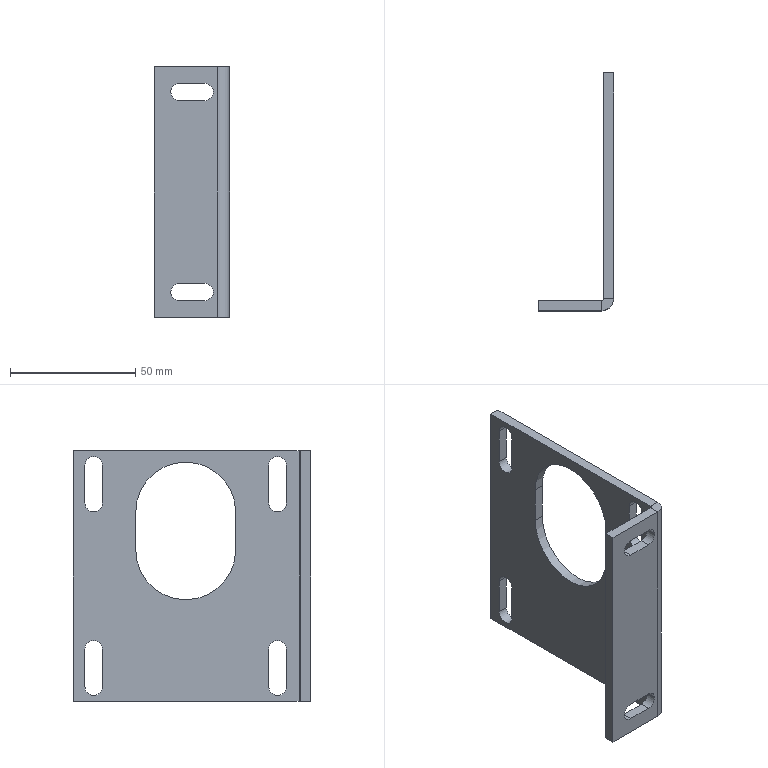Component | SolidWorks | CCD13MotorPlate-1 | 1 solid | 49 faces | volume 37340 mm3 | plane 26 | cylinder 23 | commonest cylinder face diameters 7 x18 40 x3 9.473 x1 1.473 x1